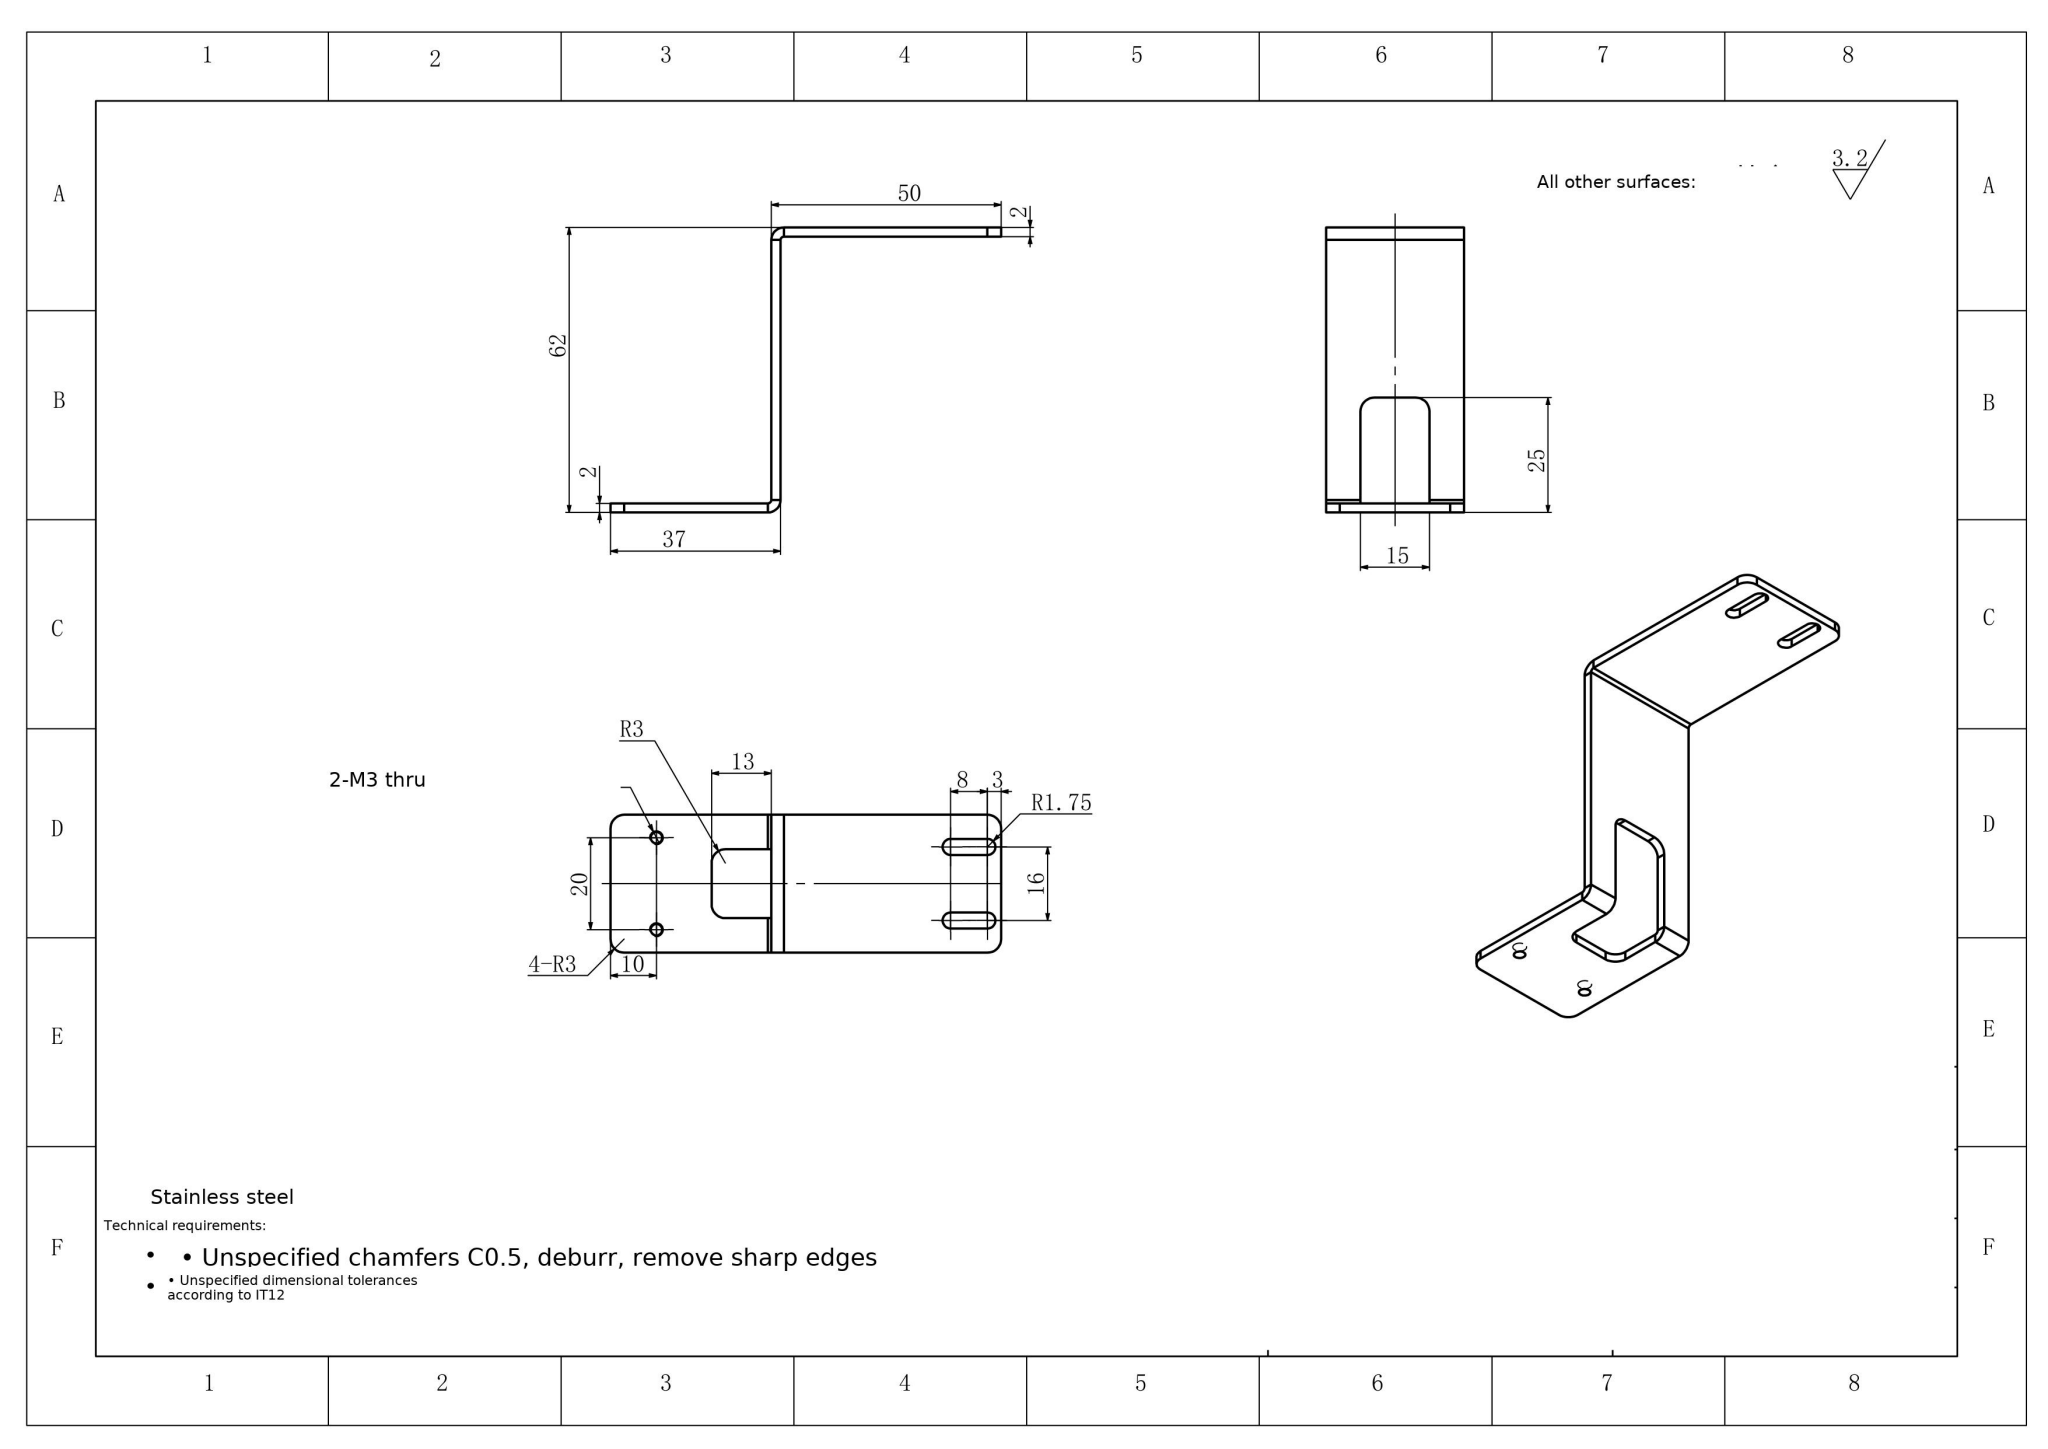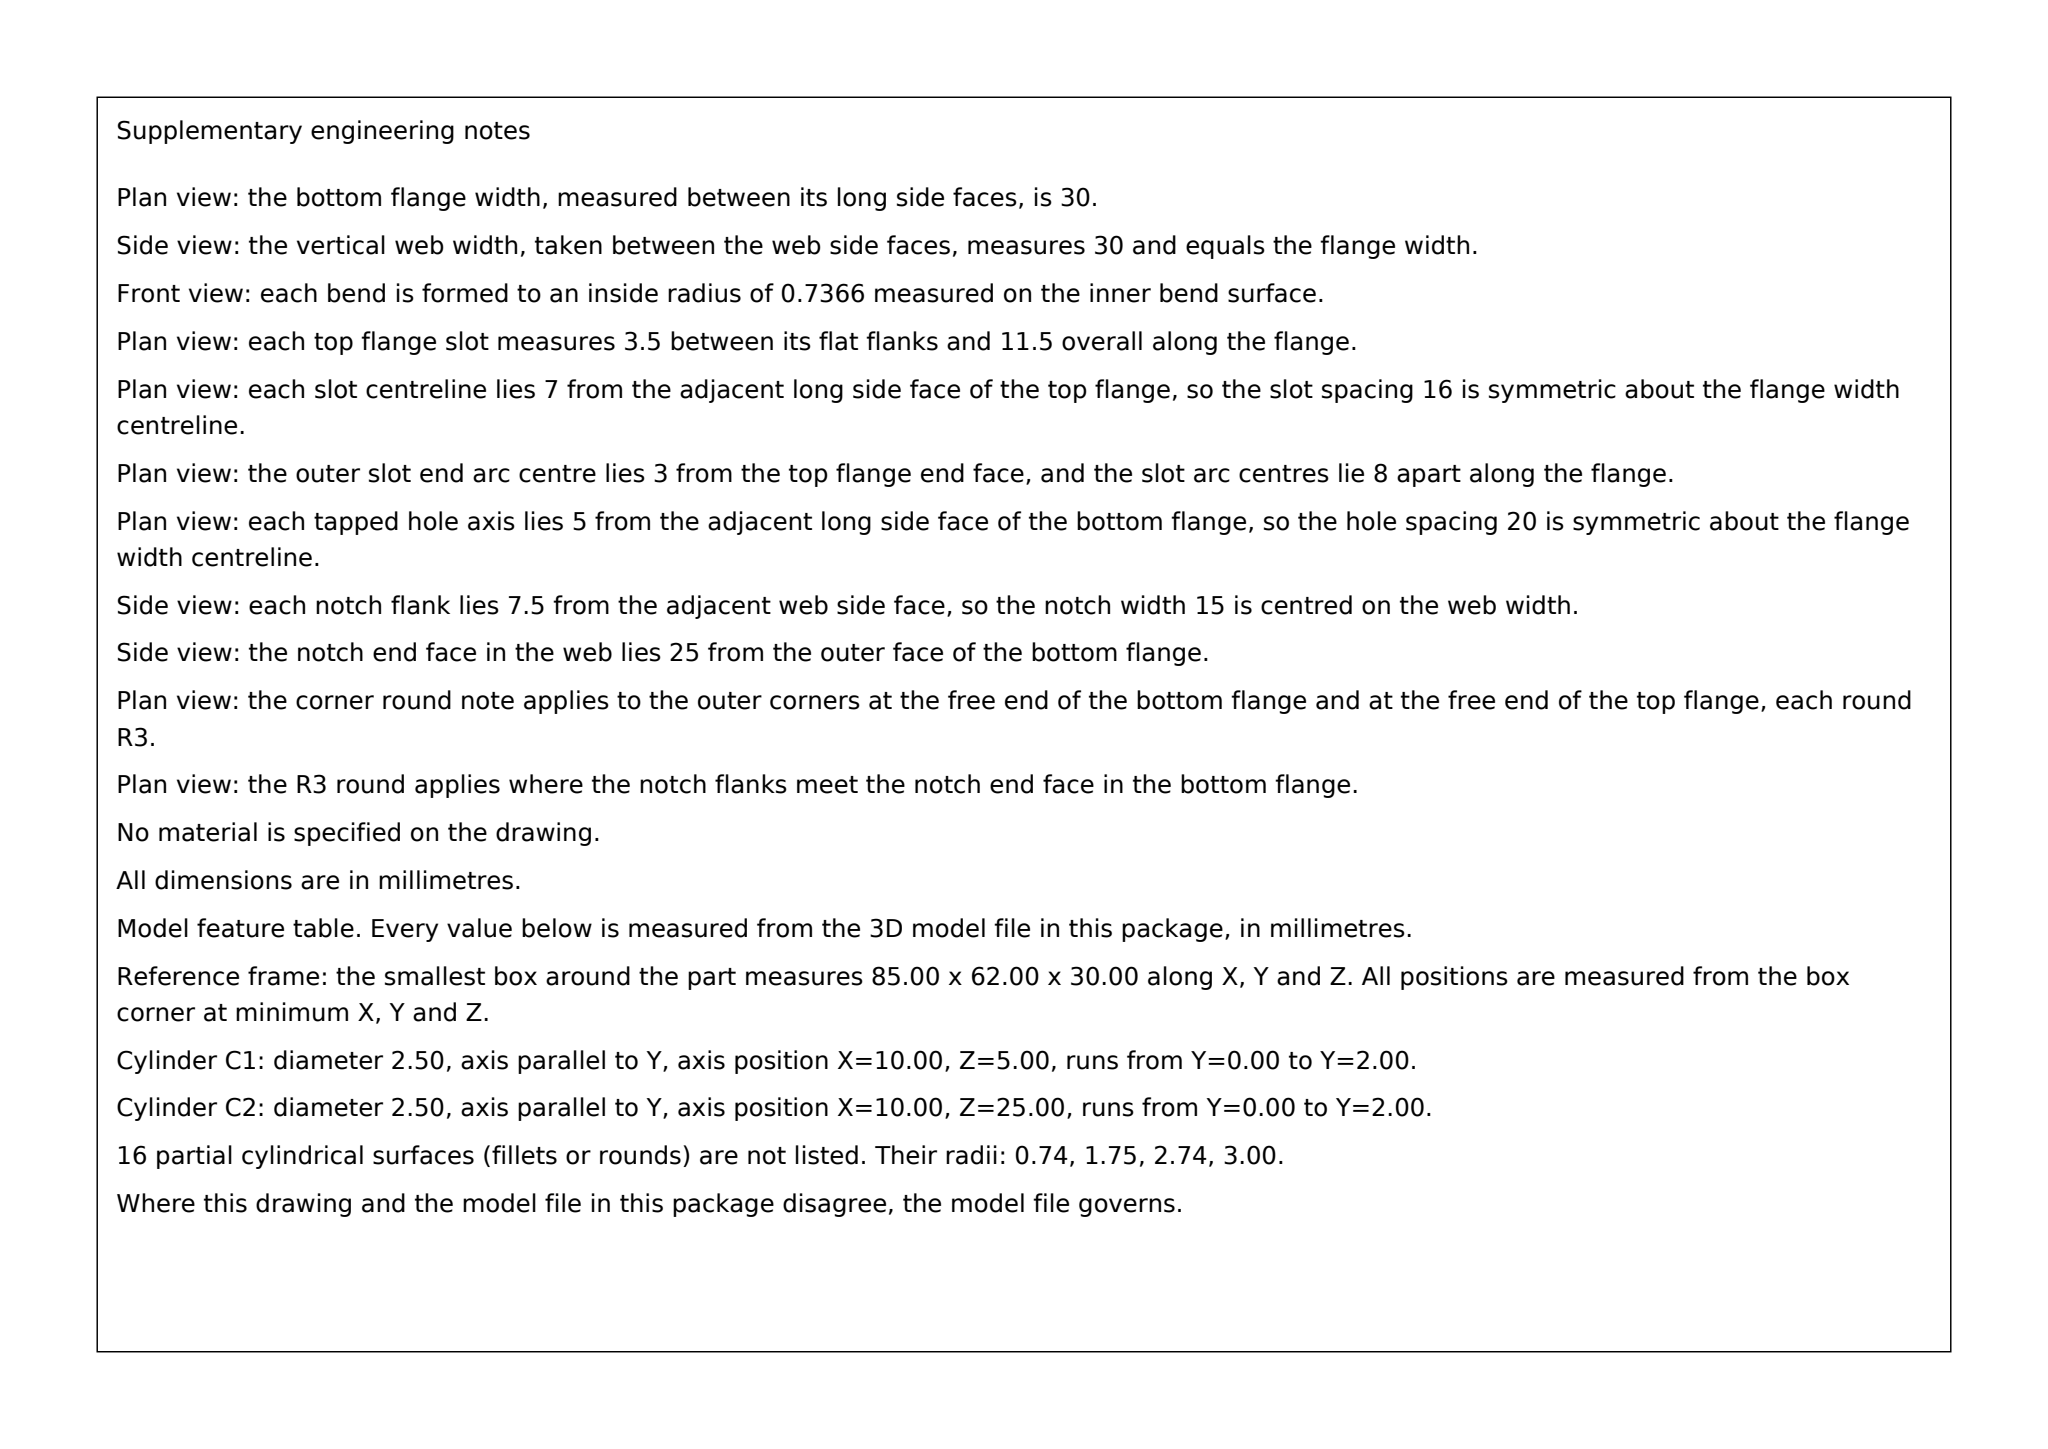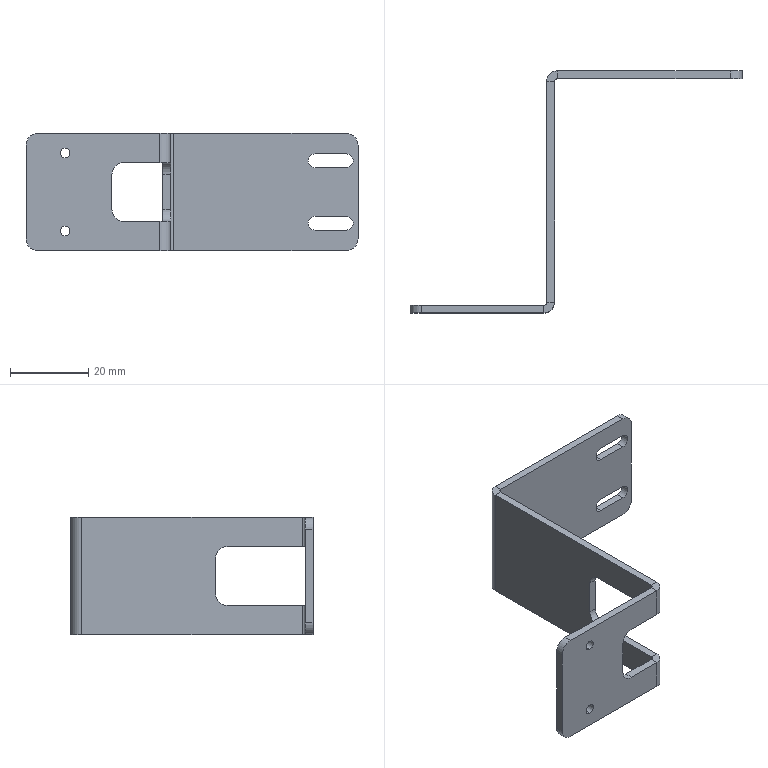Part | SolidWorks | mm | 1 solid | 52 faces | box 85 x 62 x 30 mm | volume 7323 mm3 | plane 30 | cylinder 22 | commonest cylinder face diameters 6 x8 2.5 x4 3.5 x4 1.473 x3 5.473 x3
Drawing notes:
OVERALL WIDTH 30 ACROSS STRIP, TYP ALL FLANGES | from the solid: bbox_xyz z extent = 30.0; z planes at 0.0 and 30.0
BEND RAD: R0.74 INSIDE, R2.74 OUTSIDE, 2 PL | from the solid: cyl dia 1.473 (R0.74) & 5.473 (R2.74), axis z, at [34.26,2.74] and [37.74,59.26]